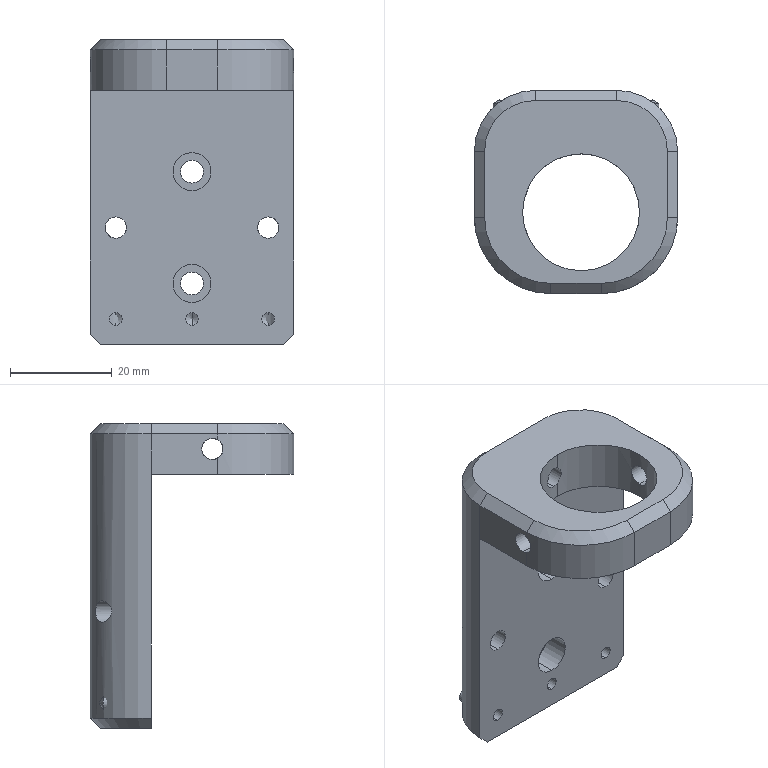Component | SolidWorks | DZ.KX.203-TC1505-20-18-05-99-1 | 1 solid | 63 faces | volume 28940 mm3 | cylinder 34 | plane 17 | cone 12 | commonest cylinder face diameters 4.2 x10 2.5 x6 7.5 x4 4.5 x4 10 x4 23 x2 30 x2 24 x2 | material Plain Carbon Steel